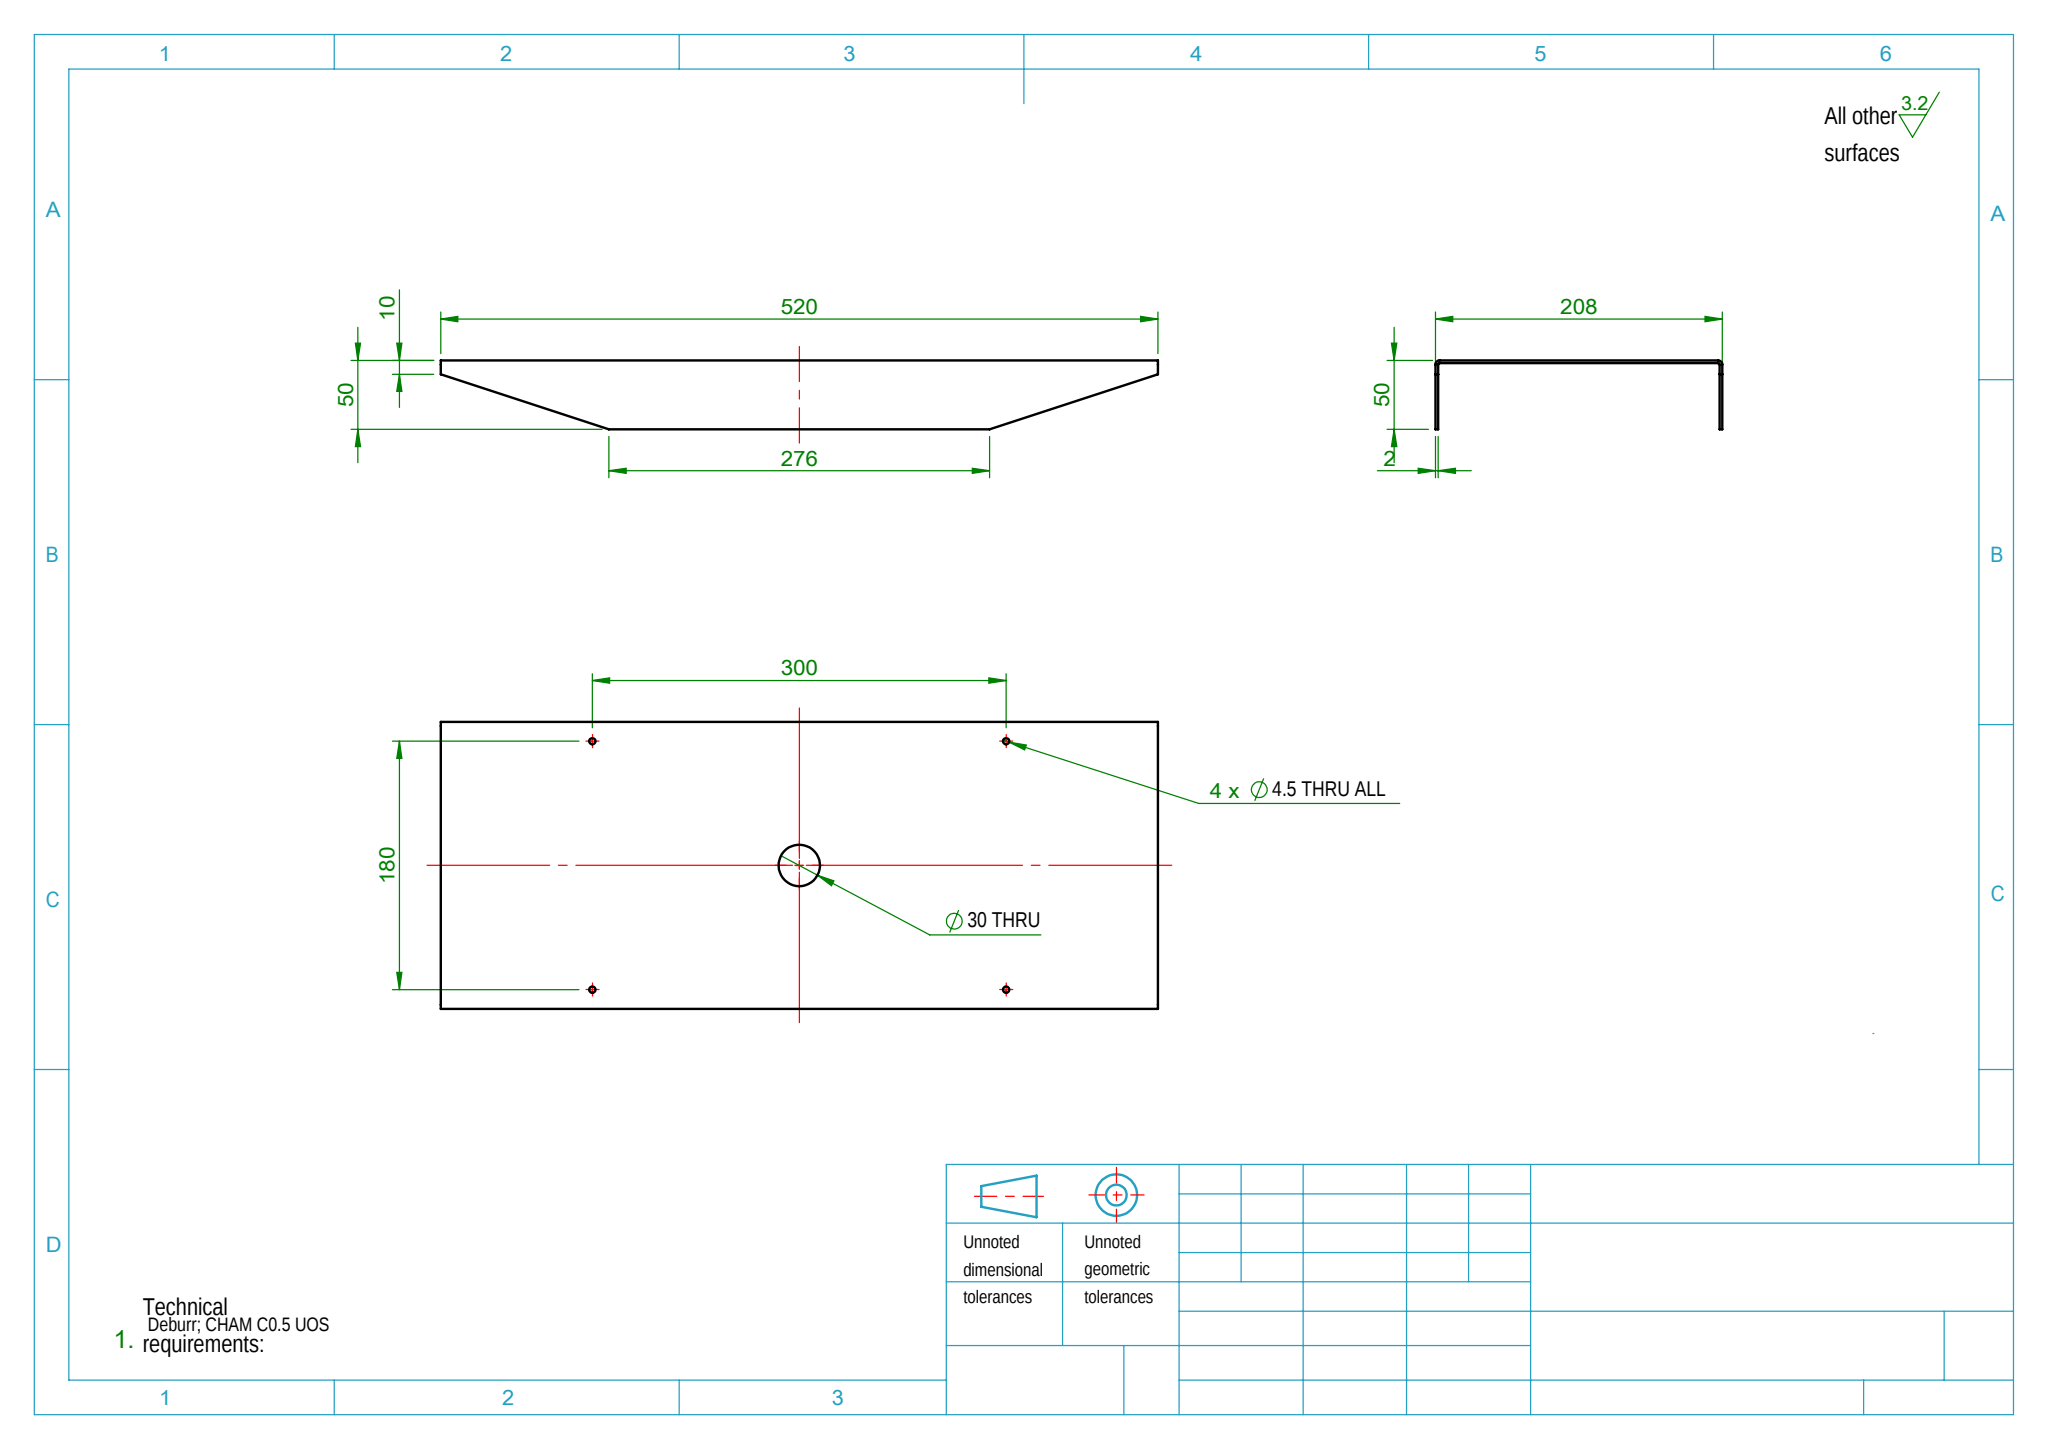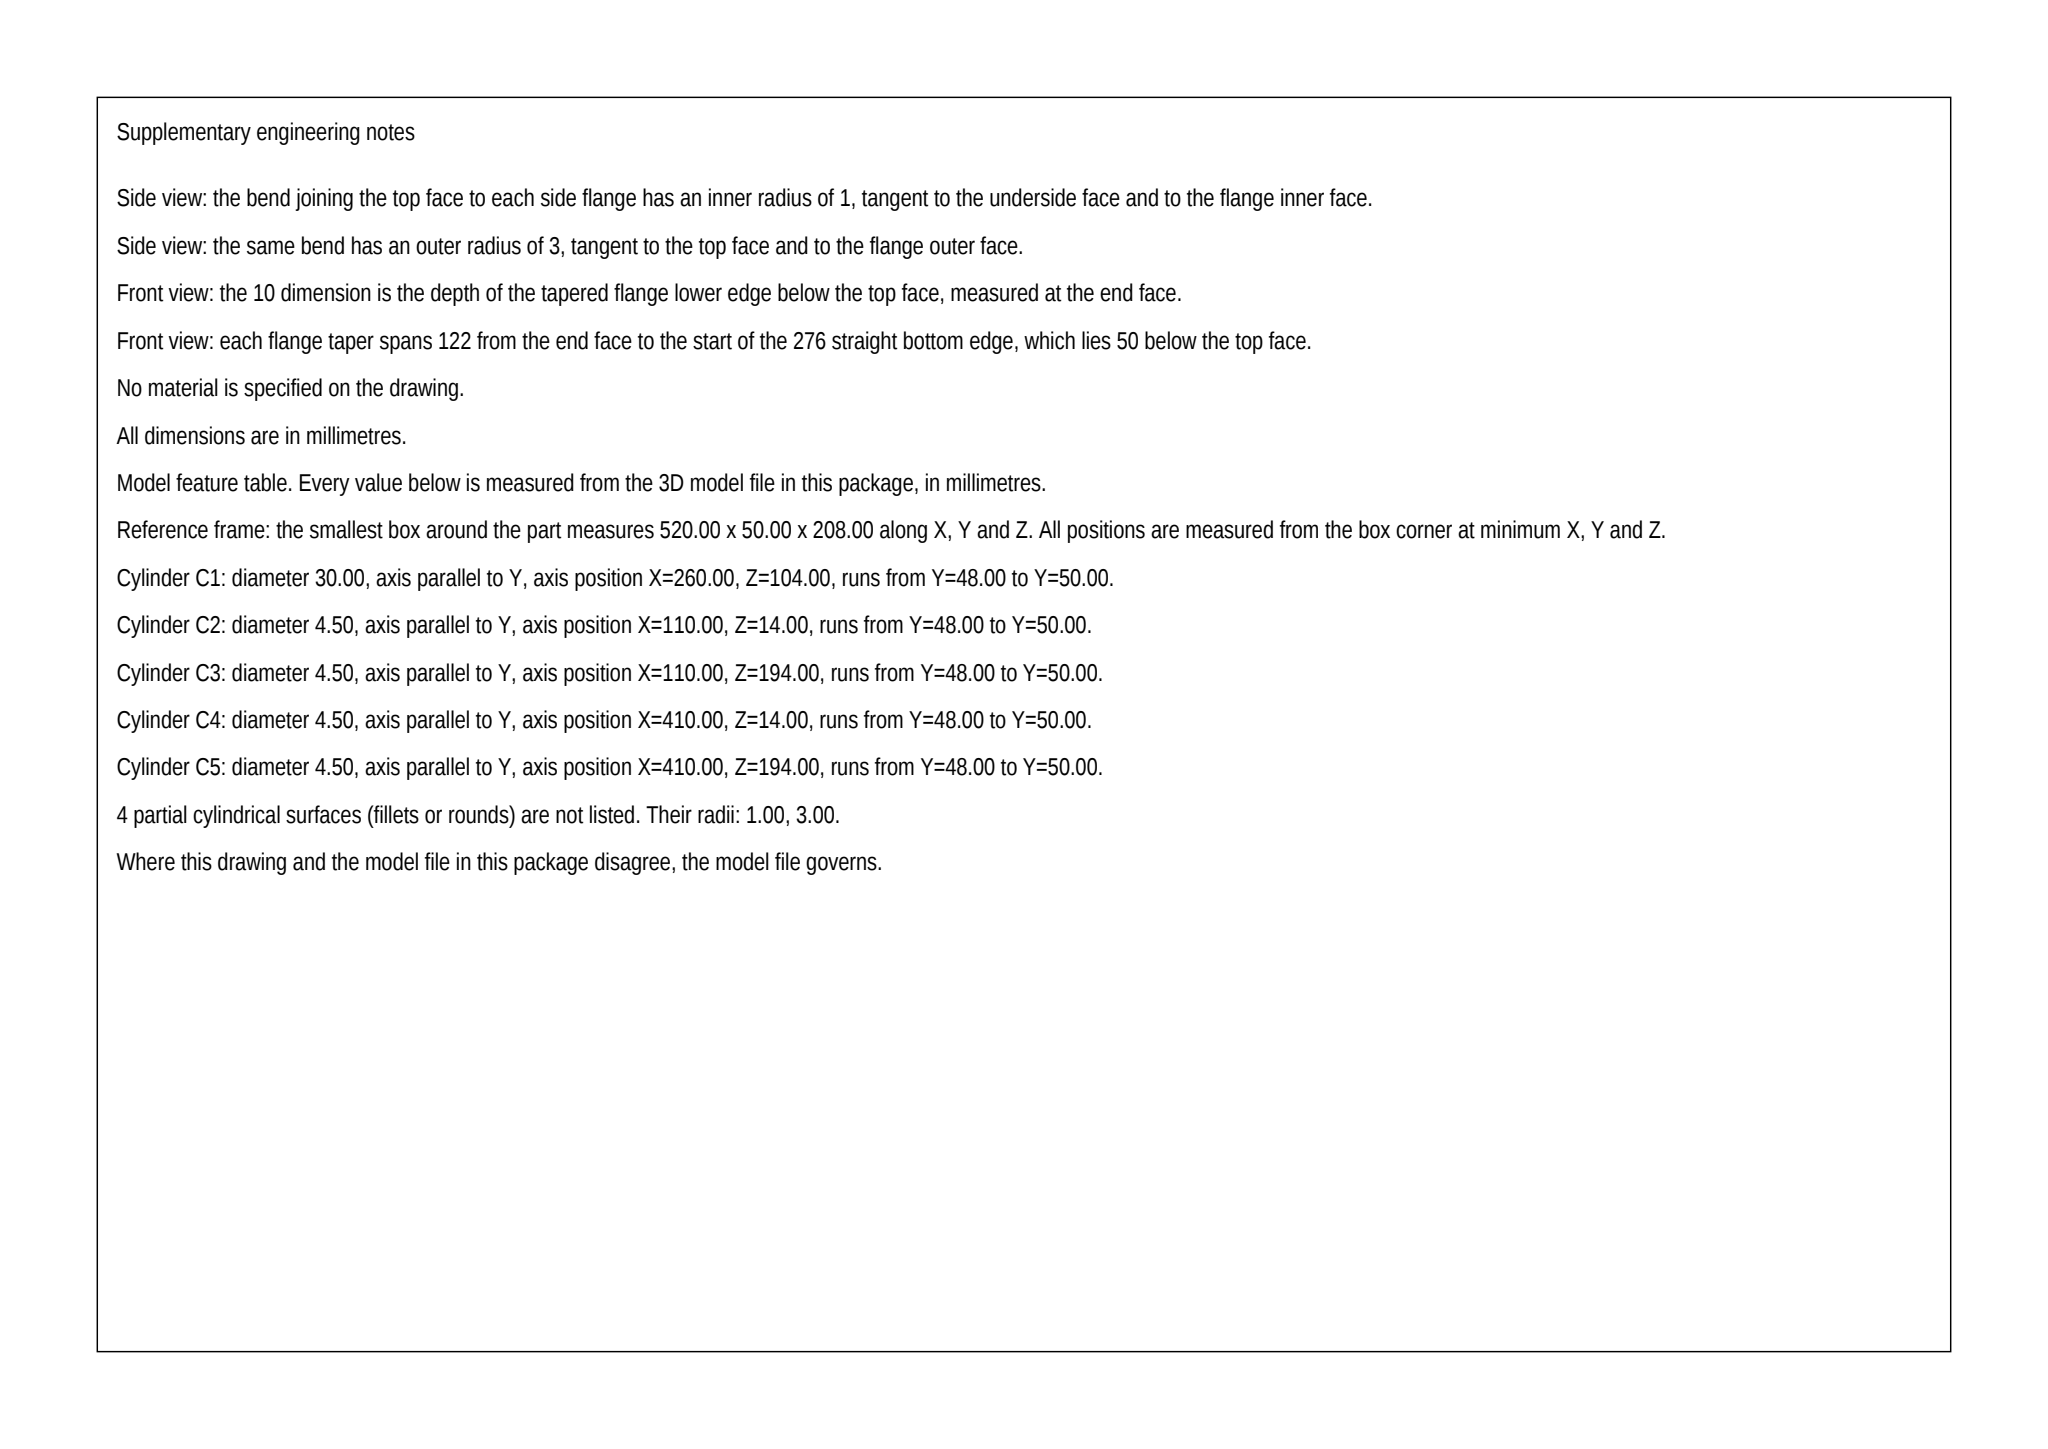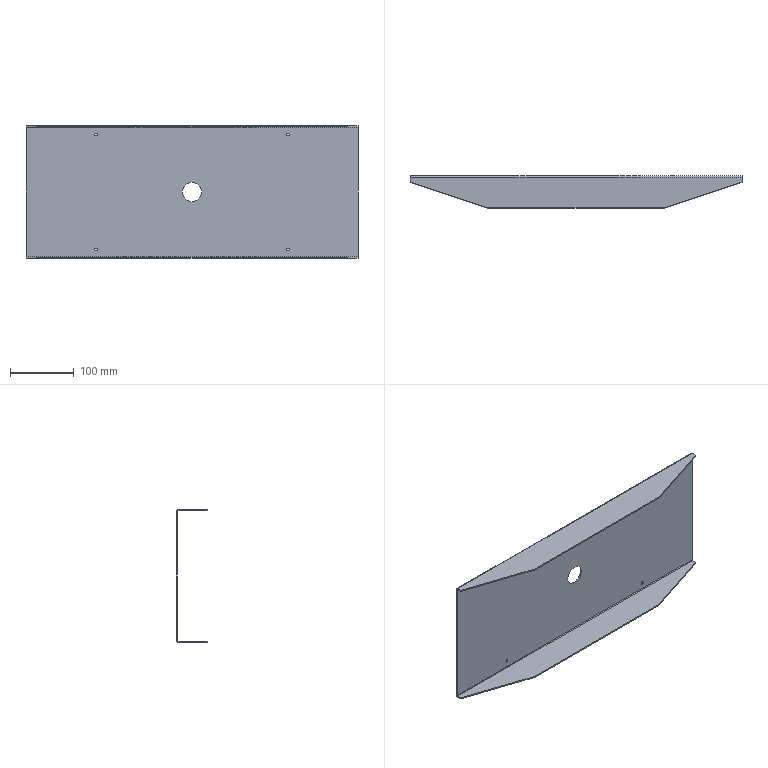Part | SolidWorks | mm | 1 solid | 36 faces | box 520 x 50 x 208 mm | volume 293314 mm3 | plane 22 | cylinder 14 | commonest cylinder face diameters 4.5 x8 30 x2 6 x2 2 x2
Drawing notes:
BEND INNER R1 TYP (OUTER R3), MATL THK 2 | from the solid: Ø2.0 x-axis cyls at y47,z3 & z205 (inner R1); Ø6.0 same axes (outer R3); y planes 48/50 give 2 thk